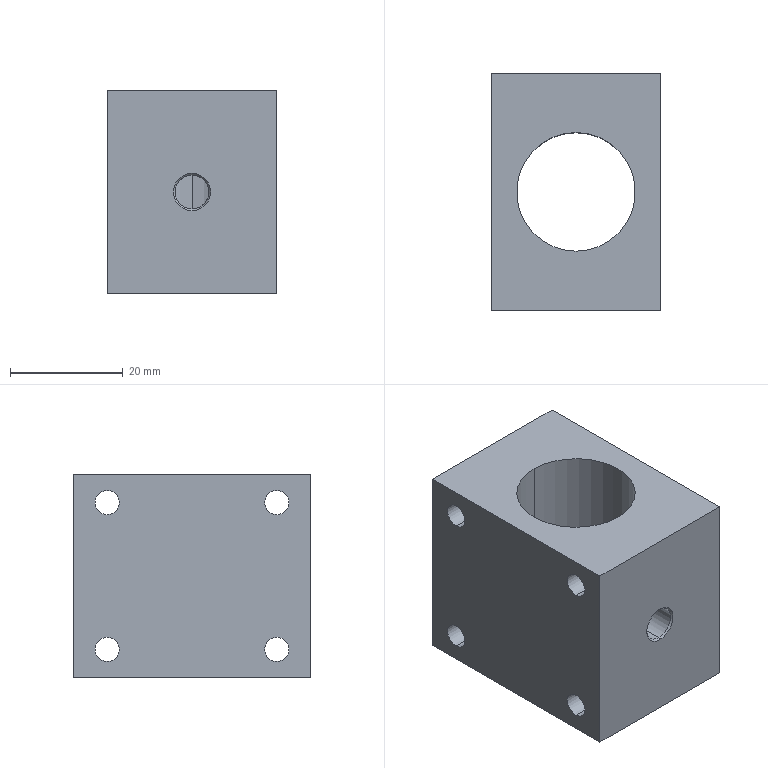Component | SolidWorks | FilmMechanism-3-1_SCLinearBearing-2 | 1 solid | 20 faces | box 30 x 42 x 36 mm | volume 30848 mm3 | cylinder 12 | plane 6 | cone 2 | commonest cylinder face diameters 4.3 x8 6 x2 21 x2
STEP:
#1=COLOUR_RGB('',0.7922,0.8196,0.9333);
#2=FILL_AREA_STYLE_COLOUR('',#1);
#3=FILL_AREA_STYLE('',(#2));
#4=SURFACE_STYLE_FILL_AREA(#3);
#5=SURFACE_SIDE_STYLE('',(#4));
#6=SURFACE_STYLE_USAGE(.BOTH.,#5);
#7=PRESENTATION_STYLE_ASSIGNMENT((#6));
#8=CARTESIAN_POINT('',(-20.718,18.334,-6.681));
#9=VERTEX_POINT('',#8);
#10=CARTESIAN_POINT('',(-20.718,18.334,-6.918));
#11=VERTEX_POINT('',#10);
#12=CARTESIAN_POINT('',(-20.718,18.334,-6.799));
#13=DIRECTION('',(0.,-1.,-0.));
#14=DIRECTION('',(0.,0.,-1.));
#15=AXIS2_PLACEMENT_3D('',#12,#13,#14);
#16=CIRCLE('',#15,0.1181);
#17=EDGE_CURVE('',#9,#11,#16,.T.);
#18=ORIENTED_EDGE('',*,*,#17,.F.);
#19=CARTESIAN_POINT('',(-20.718,18.322,-6.67));
#20=VERTEX_POINT('',#19);
#21=CARTESIAN_POINT('',(-20.718,18.322,-6.67));
#22=DIRECTION('',(0.,-0.7071,0.7071));
#23=VECTOR('',#22,39.37);
#24=LINE('',#21,#23);
#25=EDGE_CURVE('',#9,#20,#24,.T.);
#26=ORIENTED_EDGE('',*,*,#25,.T.);
#27=CARTESIAN_POINT('',(-20.718,18.322,-6.929));
#28=VERTEX_POINT('',#27);
#29=CARTESIAN_POINT('',(-20.718,18.322,-6.799));
#30=DIRECTION('',(0.,-1.,-0.));
#31=DIRECTION('',(0.,0.,-1.));
#32=AXIS2_PLACEMENT_3D('',#29,#30,#31);
#33=CIRCLE('',#32,0.1299);
#34=EDGE_CURVE('',#20,#28,#33,.T.);
#35=ORIENTED_EDGE('',*,*,#34,.T.);
#36=CARTESIAN_POINT('',(-20.718,18.322,-6.929));
#37=DIRECTION('',(0.,-0.7071,-0.7071));
#38=VECTOR('',#37,39.37);
#39=LINE('',#36,#38);
#40=EDGE_CURVE('',#11,#28,#39,.T.);
#41=ORIENTED_EDGE('',*,*,#40,.F.);
#42=EDGE_LOOP('',(#18,#26,#35,#41));
#43=FACE_OUTER_BOUND('',#42,.T.);
#44=CARTESIAN_POINT('',(-20.718,18.322,-6.799));
#45=DIRECTION('',(0.,-1.,-0.));
#46=DIRECTION('',(0.,0.,-1.));
#47=AXIS2_PLACEMENT_3D('',#44,#45,#46);
#48=CONICAL_SURFACE('',#47,0.1299,0.7854);
#49=ADVANCED_FACE('',(#43),#48,.F.);
#50=CARTESIAN_POINT('',(-20.718,18.735,-6.681));
#51=VERTEX_POINT('',#50);
#52=CARTESIAN_POINT('',(-20.718,18.735,-6.918));
#53=VERTEX_POINT('',#52);
#54=CARTESIAN_POINT('',(-20.718,18.735,-6.681));
#55=CARTESIAN_POINT('',(-20.726,18.735,-6.681));
#56=CARTESIAN_POINT('',(-20.734,18.735,-6.682));
#57=CARTESIAN_POINT('',(-20.749,18.736,-6.685));
#58=CARTESIAN_POINT('',(-20.757,18.737,-6.687));
#59=CARTESIAN_POINT('',(-20.771,18.738,-6.693));
#60=CARTESIAN_POINT('',(-20.778,18.739,-6.697));
#61=CARTESIAN_POINT('',(-20.79,18.741,-6.706));
#62=CARTESIAN_POINT('',(-20.796,18.743,-6.71));
#63=CARTESIAN_POINT('',(-20.807,18.745,-6.721));
#64=CARTESIAN_POINT('',(-20.812,18.746,-6.727));
#65=CARTESIAN_POINT('',(-20.821,18.748,-6.74));
#66=CARTESIAN_POINT('',(-20.824,18.749,-6.747));
#67=CARTESIAN_POINT('',(-20.83,18.751,-6.761));
#68=CARTESIAN_POINT('',(-20.833,18.751,-6.769));
#69=CARTESIAN_POINT('',(-20.836,18.752,-6.784));
#70=CARTESIAN_POINT('',(-20.836,18.752,-6.792));
#71=CARTESIAN_POINT('',(-20.836,18.752,-6.807));
#72=CARTESIAN_POINT('',(-20.836,18.752,-6.815));
#73=CARTESIAN_POINT('',(-20.833,18.751,-6.83));
#74=CARTESIAN_POINT('',(-20.83,18.751,-6.838));
#75=CARTESIAN_POINT('',(-20.822,18.748,-6.859));
#76=CARTESIAN_POINT('',(-20.813,18.746,-6.872));
#77=CARTESIAN_POINT('',(-20.797,18.743,-6.888));
#78=CARTESIAN_POINT('',(-20.79,18.741,-6.893));
#79=CARTESIAN_POINT('',(-20.778,18.739,-6.902));
#80=CARTESIAN_POINT('',(-20.771,18.738,-6.906));
#81=CARTESIAN_POINT('',(-20.757,18.737,-6.911));
#82=CARTESIAN_POINT('',(-20.749,18.736,-6.914));
#83=CARTESIAN_POINT('',(-20.734,18.735,-6.917));
#84=CARTESIAN_POINT('',(-20.726,18.735,-6.918));
#85=CARTESIAN_POINT('',(-20.718,18.735,-6.918));
#86=B_SPLINE_CURVE_WITH_KNOTS('',3,(#54,#55,#56,#57,#58,#59,#60,#61,#62,#63,#64,#65,#66,#67,#68,#69,#70,#71,#72,#73,#74,#75,#76,#77,#78,#79,#80,#81,#82,#83,#84,#85),.UNSPECIFIED.,.F.,.F.,(4,2,2,2,2,2,2,2,2,2,2,2,2,2,2,4),(0.009429,0.01002,0.01061,0.0112,0.01179,0.01237,0.01296,0.01355,0.01414,0.01473,0.01532,0.0165,0.01709,0.01768,0.01827,0.01885),.UNSPECIFIED.);
#87=EDGE_CURVE('',#51,#53,#86,.T.);
#88=ORIENTED_EDGE('',*,*,#87,.F.);
#89=CARTESIAN_POINT('',(-20.718,18.322,-6.681));
#90=DIRECTION('',(0.,-1.,-0.));
#91=VECTOR('',#90,39.37);
#92=LINE('',#89,#91);
#93=EDGE_CURVE('',#51,#9,#92,.T.);
#94=ORIENTED_EDGE('',*,*,#93,.T.);
#95=ORIENTED_EDGE('',*,*,#17,.T.);
#96=CARTESIAN_POINT('',(-20.718,18.322,-6.918));
#97=DIRECTION('',(0.,-1.,-0.));
#98=VECTOR('',#97,39.37);
#99=LINE('',#96,#98);
#100=EDGE_CURVE('',#53,#11,#99,.T.);
#101=ORIENTED_EDGE('',*,*,#100,.F.);
#102=EDGE_LOOP('',(#88,#94,#95,#101));
#103=FACE_OUTER_BOUND('',#102,.T.);
#104=CARTESIAN_POINT('',(-20.718,18.322,-6.799));
#105=DIRECTION('',(0.,-1.,-0.));
#106=DIRECTION('',(0.,0.,-1.));
#107=AXIS2_PLACEMENT_3D('',#104,#105,#106);
#108=CYLINDRICAL_SURFACE('',#107,0.1181);
#109=ADVANCED_FACE('',(#103),#108,.F.);
#110=CARTESIAN_POINT('',(-20.718,19.562,-7.508));
#111=VERTEX_POINT('',#110);
#112=CARTESIAN_POINT('',(-20.718,18.735,-7.508));
#113=VERTEX_POINT('',#112);
#114=CARTESIAN_POINT('',(-20.718,19.149,-7.508));
#115=DIRECTION('',(-0.,-0.,1.));
#116=DIRECTION('',(0.,-1.,-0.));
#117=AXIS2_PLACEMENT_3D('',#114,#115,#116);
#118=CIRCLE('',#117,0.4134);
#119=EDGE_CURVE('',#111,#113,#118,.T.);
#120=ORIENTED_EDGE('',*,*,#119,.F.);
#121=CARTESIAN_POINT('',(-20.718,19.562,-6.091));
#122=VERTEX_POINT('',#121);
#123=CARTESIAN_POINT('',(-20.718,19.562,-6.091));
#124=DIRECTION('',(-0.,-0.,1.));
#125=VECTOR('',#124,39.37);
#126=LINE('',#123,#125);
#127=EDGE_CURVE('',#111,#122,#126,.T.);
#128=ORIENTED_EDGE('',*,*,#127,.T.);
#129=CARTESIAN_POINT('',(-20.718,18.735,-6.091));
#130=VERTEX_POINT('',#129);
#131=CARTESIAN_POINT('',(-20.718,19.149,-6.091));
#132=DIRECTION('',(-0.,-0.,1.));
#133=DIRECTION('',(0.,-1.,-0.));
#134=AXIS2_PLACEMENT_3D('',#131,#132,#133);
#135=CIRCLE('',#134,0.4134);
#136=EDGE_CURVE('',#122,#130,#135,.T.);
#137=ORIENTED_EDGE('',*,*,#136,.T.);
#138=CARTESIAN_POINT('',(-20.718,18.735,-6.091));
#139=DIRECTION('',(-0.,-0.,1.));
#140=VECTOR('',#139,39.37);
#141=LINE('',#138,#140);
#142=EDGE_CURVE('',#51,#130,#141,.T.);
#143=ORIENTED_EDGE('',*,*,#142,.F.);
#144=ORIENTED_EDGE('',*,*,#87,.T.);
#145=CARTESIAN_POINT('',(-20.718,18.735,-6.091));
#146=DIRECTION('',(-0.,-0.,1.));
#147=VECTOR('',#146,39.37);
#148=LINE('',#145,#147);
#149=EDGE_CURVE('',#113,#53,#148,.T.);
#150=ORIENTED_EDGE('',*,*,#149,.F.);
#151=EDGE_LOOP('',(#120,#128,#137,#143,#144,#150));
#152=FACE_OUTER_BOUND('',#151,.T.);
#153=CARTESIAN_POINT('',(-20.718,19.149,-6.091));
#154=DIRECTION('',(-0.,-0.,1.));
#155=DIRECTION('',(0.,-1.,-0.));
#156=AXIS2_PLACEMENT_3D('',#153,#154,#155);
#157=CYLINDRICAL_SURFACE('',#156,0.4134);
#158=ADVANCED_FACE('',(#152),#157,.F.);
#159=CARTESIAN_POINT('',(-20.128,19.739,-7.227));
#160=VERTEX_POINT('',#159);
#161=CARTESIAN_POINT('',(-20.128,19.739,-7.396));
#162=VERTEX_POINT('',#161);
#163=CARTESIAN_POINT('',(-20.128,19.739,-7.311));
#164=DIRECTION('',(-1.,-0.,-0.));
#165=DIRECTION('',(0.,0.,-1.));
#166=AXIS2_PLACEMENT_3D('',#163,#164,#165);
#167=CIRCLE('',#166,0.08465);
#168=EDGE_CURVE('',#160,#162,#167,.T.);
#169=ORIENTED_EDGE('',*,*,#168,.F.);
#170=CARTESIAN_POINT('',(-21.309,19.739,-7.227));
#171=VERTEX_POINT('',#170);
#172=CARTESIAN_POINT('',(-21.309,19.739,-7.227));
#173=DIRECTION('',(-1.,-0.,-0.));
#174=VECTOR('',#173,39.37);
#175=LINE('',#172,#174);
#176=EDGE_CURVE('',#160,#171,#175,.T.);
#177=ORIENTED_EDGE('',*,*,#176,.T.);
#178=CARTESIAN_POINT('',(-21.309,19.739,-7.396));
#179=VERTEX_POINT('',#178);
#180=CARTESIAN_POINT('',(-21.309,19.739,-7.311));
#181=DIRECTION('',(-1.,-0.,-0.));
#182=DIRECTION('',(0.,0.,-1.));
#183=AXIS2_PLACEMENT_3D('',#180,#181,#182);
#184=CIRCLE('',#183,0.08465);
#185=EDGE_CURVE('',#171,#179,#184,.T.);
#186=ORIENTED_EDGE('',*,*,#185,.T.);
#187=CARTESIAN_POINT('',(-21.309,19.739,-7.396));
#188=DIRECTION('',(-1.,-0.,-0.));
#189=VECTOR('',#188,39.37);
#190=LINE('',#187,#189);
#191=EDGE_CURVE('',#162,#179,#190,.T.);
#192=ORIENTED_EDGE('',*,*,#191,.F.);
#193=EDGE_LOOP('',(#169,#177,#186,#192));
#194=FACE_OUTER_BOUND('',#193,.T.);
#195=CARTESIAN_POINT('',(-21.309,19.739,-7.311));
#196=DIRECTION('',(-1.,-0.,-0.));
#197=DIRECTION('',(0.,0.,-1.));
#198=AXIS2_PLACEMENT_3D('',#195,#196,#197);
#199=CYLINDRICAL_SURFACE('',#198,0.08465);
#200=ADVANCED_FACE('',(#194),#199,.F.);
#201=CARTESIAN_POINT('',(-20.128,19.739,-6.203));
#202=VERTEX_POINT('',#201);
#203=CARTESIAN_POINT('',(-20.128,19.739,-6.372));
#204=VERTEX_POINT('',#203);
#205=CARTESIAN_POINT('',(-20.128,19.739,-6.288));
#206=DIRECTION('',(-1.,-0.,-0.));
#207=DIRECTION('',(0.,0.,-1.));
#208=AXIS2_PLACEMENT_3D('',#205,#206,#207);
#209=CIRCLE('',#208,0.08465);
#210=EDGE_CURVE('',#202,#204,#209,.T.);
#211=ORIENTED_EDGE('',*,*,#210,.F.);
#212=CARTESIAN_POINT('',(-21.309,19.739,-6.203));
#213=VERTEX_POINT('',#212);
#214=CARTESIAN_POINT('',(-21.309,19.739,-6.203));
#215=DIRECTION('',(-1.,-0.,-0.));
#216=VECTOR('',#215,39.37);
#217=LINE('',#214,#216);
#218=EDGE_CURVE('',#202,#213,#217,.T.);
#219=ORIENTED_EDGE('',*,*,#218,.T.);
#220=CARTESIAN_POINT('',(-21.309,19.739,-6.372));
#221=VERTEX_POINT('',#220);
#222=CARTESIAN_POINT('',(-21.309,19.739,-6.288));
#223=DIRECTION('',(-1.,-0.,-0.));
#224=DIRECTION('',(0.,0.,-1.));
#225=AXIS2_PLACEMENT_3D('',#222,#223,#224);
#226=CIRCLE('',#225,0.08465);
#227=EDGE_CURVE('',#213,#221,#226,.T.);
#228=ORIENTED_EDGE('',*,*,#227,.T.);
#229=CARTESIAN_POINT('',(-21.309,19.739,-6.372));
#230=DIRECTION('',(-1.,-0.,-0.));
#231=VECTOR('',#230,39.37);
#232=LINE('',#229,#231);
#233=EDGE_CURVE('',#204,#221,#232,.T.);
#234=ORIENTED_EDGE('',*,*,#233,.F.);
#235=EDGE_LOOP('',(#211,#219,#228,#234));
#236=FACE_OUTER_BOUND('',#235,.T.);
#237=CARTESIAN_POINT('',(-21.309,19.739,-6.288));
#238=DIRECTION('',(-1.,-0.,-0.));
#239=DIRECTION('',(0.,0.,-1.));
#240=AXIS2_PLACEMENT_3D('',#237,#238,#239);
#241=CYLINDRICAL_SURFACE('',#240,0.08465);
#242=ADVANCED_FACE('',(#236),#241,.F.);
#243=CARTESIAN_POINT('',(-20.128,18.558,-7.227));
#244=VERTEX_POINT('',#243);
#245=CARTESIAN_POINT('',(-20.128,18.558,-7.396));
#246=VERTEX_POINT('',#245);
#247=CARTESIAN_POINT('',(-20.128,18.558,-7.311));
#248=DIRECTION('',(-1.,-0.,-0.));
#249=DIRECTION('',(0.,0.,-1.));
#250=AXIS2_PLACEMENT_3D('',#247,#248,#249);
#251=CIRCLE('',#250,0.08465);
#252=EDGE_CURVE('',#244,#246,#251,.T.);
#253=ORIENTED_EDGE('',*,*,#252,.F.);
#254=CARTESIAN_POINT('',(-21.309,18.558,-7.227));
#255=VERTEX_POINT('',#254);
#256=CARTESIAN_POINT('',(-21.309,18.558,-7.227));
#257=DIRECTION('',(-1.,-0.,-0.));
#258=VECTOR('',#257,39.37);
#259=LINE('',#256,#258);
#260=EDGE_CURVE('',#244,#255,#259,.T.);
#261=ORIENTED_EDGE('',*,*,#260,.T.);
#262=CARTESIAN_POINT('',(-21.309,18.558,-7.396));
#263=VERTEX_POINT('',#262);
#264=CARTESIAN_POINT('',(-21.309,18.558,-7.311));
#265=DIRECTION('',(-1.,-0.,-0.));
#266=DIRECTION('',(0.,0.,-1.));
#267=AXIS2_PLACEMENT_3D('',#264,#265,#266);
#268=CIRCLE('',#267,0.08465);
#269=EDGE_CURVE('',#255,#263,#268,.T.);
#270=ORIENTED_EDGE('',*,*,#269,.T.);
#271=CARTESIAN_POINT('',(-21.309,18.558,-7.396));
#272=DIRECTION('',(-1.,-0.,-0.));
#273=VECTOR('',#272,39.37);
#274=LINE('',#271,#273);
#275=EDGE_CURVE('',#246,#263,#274,.T.);
#276=ORIENTED_EDGE('',*,*,#275,.F.);
#277=EDGE_LOOP('',(#253,#261,#270,#276));
#278=FACE_OUTER_BOUND('',#277,.T.);
#279=CARTESIAN_POINT('',(-21.309,18.558,-7.311));
#280=DIRECTION('',(-1.,-0.,-0.));
#281=DIRECTION('',(0.,0.,-1.));
#282=AXIS2_PLACEMENT_3D('',#279,#280,#281);
#283=CYLINDRICAL_SURFACE('',#282,0.08465);
#284=ADVANCED_FACE('',(#278),#283,.F.);
#285=CARTESIAN_POINT('',(-20.128,18.558,-6.203));
#286=VERTEX_POINT('',#285);
#287=CARTESIAN_POINT('',(-20.128,18.558,-6.372));
#288=VERTEX_POINT('',#287);
#289=CARTESIAN_POINT('',(-20.128,18.558,-6.288));
#290=DIRECTION('',(-1.,-0.,-0.));
#291=DIRECTION('',(0.,0.,-1.));
#292=AXIS2_PLACEMENT_3D('',#289,#290,#291);
#293=CIRCLE('',#292,0.08465);
#294=EDGE_CURVE('',#286,#288,#293,.T.);
#295=ORIENTED_EDGE('',*,*,#294,.F.);
#296=CARTESIAN_POINT('',(-21.309,18.558,-6.203));
#297=VERTEX_POINT('',#296);
#298=CARTESIAN_POINT('',(-21.309,18.558,-6.203));
#299=DIRECTION('',(-1.,-0.,-0.));
#300=VECTOR('',#299,39.37);
#301=LINE('',#298,#300);
#302=EDGE_CURVE('',#286,#297,#301,.T.);
#303=ORIENTED_EDGE('',*,*,#302,.T.);
#304=CARTESIAN_POINT('',(-21.309,18.558,-6.372));
#305=VERTEX_POINT('',#304);
#306=CARTESIAN_POINT('',(-21.309,18.558,-6.288));
#307=DIRECTION('',(-1.,-0.,-0.));
#308=DIRECTION('',(0.,0.,-1.));
#309=AXIS2_PLACEMENT_3D('',#306,#307,#308);
#310=CIRCLE('',#309,0.08465);
#311=EDGE_CURVE('',#297,#305,#310,.T.);
#312=ORIENTED_EDGE('',*,*,#311,.T.);
#313=CARTESIAN_POINT('',(-21.309,18.558,-6.372));
#314=DIRECTION('',(-1.,-0.,-0.));
#315=VECTOR('',#314,39.37);
#316=LINE('',#313,#315);
#317=EDGE_CURVE('',#288,#305,#316,.T.);
#318=ORIENTED_EDGE('',*,*,#317,.F.);
#319=EDGE_LOOP('',(#295,#303,#312,#318));
#320=FACE_OUTER_BOUND('',#319,.T.);
#321=CARTESIAN_POINT('',(-21.309,18.558,-6.288));
#322=DIRECTION('',(-1.,-0.,-0.));
#323=DIRECTION('',(0.,0.,-1.));
#324=AXIS2_PLACEMENT_3D('',#321,#322,#323);
#325=CYLINDRICAL_SURFACE('',#324,0.08465);
#326=ADVANCED_FACE('',(#320),#325,.F.);
#327=CARTESIAN_POINT('',(-20.718,18.322,-6.799));
#328=DIRECTION('',(0.,-1.,-0.));
#329=DIRECTION('',(0.,0.,-1.));
#330=AXIS2_PLACEMENT_3D('',#327,#328,#329);
#331=CIRCLE('',#330,0.1299);
#332=EDGE_CURVE('',#28,#20,#331,.T.);
#333=ORIENTED_EDGE('',*,*,#332,.F.);
#334=ORIENTED_EDGE('',*,*,#34,.F.);
#335=EDGE_LOOP('',(#333,#334));
#336=FACE_BOUND('',#335,.T.);
#337=CARTESIAN_POINT('',(-21.309,18.322,-7.508));
#338=VERTEX_POINT('',#337);
#339=CARTESIAN_POINT('',(-21.309,18.322,-6.091));
#340=VERTEX_POINT('',#339);
#341=CARTESIAN_POINT('',(-21.309,18.322,-7.508));
#342=DIRECTION('',(-0.,-0.,1.));
#343=VECTOR('',#342,39.37);
#344=LINE('',#341,#343);
#345=EDGE_CURVE('',#338,#340,#344,.T.);
#346=ORIENTED_EDGE('',*,*,#345,.F.);
#347=CARTESIAN_POINT('',(-20.128,18.322,-7.508));
#348=VERTEX_POINT('',#347);
#349=CARTESIAN_POINT('',(-20.128,18.322,-7.508));
#350=DIRECTION('',(-1.,-0.,-0.));
#351=VECTOR('',#350,39.37);
#352=LINE('',#349,#351);
#353=EDGE_CURVE('',#348,#338,#352,.T.);
#354=ORIENTED_EDGE('',*,*,#353,.F.);
#355=CARTESIAN_POINT('',(-20.128,18.322,-6.091));
#356=VERTEX_POINT('',#355);
#357=CARTESIAN_POINT('',(-20.128,18.322,-7.508));
#358=DIRECTION('',(-0.,-0.,1.));
#359=VECTOR('',#358,39.37);
#360=LINE('',#357,#359);
#361=EDGE_CURVE('',#348,#356,#360,.T.);
#362=ORIENTED_EDGE('',*,*,#361,.T.);
#363=CARTESIAN_POINT('',(-20.128,18.322,-6.091));
#364=DIRECTION('',(-1.,-0.,-0.));
#365=VECTOR('',#364,39.37);
#366=LINE('',#363,#365);
#367=EDGE_CURVE('',#356,#340,#366,.T.);
#368=ORIENTED_EDGE('',*,*,#367,.T.);
#369=EDGE_LOOP('',(#346,#354,#362,#368));
#370=FACE_OUTER_BOUND('',#369,.T.);
#371=CARTESIAN_POINT('',(-20.128,18.322,-7.508));
#372=DIRECTION('',(0.,-1.,-0.));
#373=DIRECTION('',(0.,0.,-1.));
#374=AXIS2_PLACEMENT_3D('',#371,#372,#373);
#375=PLANE('',#374);
#376=ADVANCED_FACE('',(#336,#370),#375,.T.);
#377=CARTESIAN_POINT('',(-20.718,19.149,-7.508));
#378=DIRECTION('',(-0.,-0.,1.));
#379=DIRECTION('',(0.,-1.,-0.));
#380=AXIS2_PLACEMENT_3D('',#377,#378,#379);
#381=CIRCLE('',#380,0.4134);
#382=EDGE_CURVE('',#113,#111,#381,.T.);
#383=ORIENTED_EDGE('',*,*,#382,.T.);
#384=ORIENTED_EDGE('',*,*,#119,.T.);
#385=EDGE_LOOP('',(#383,#384));
#386=FACE_BOUND('',#385,.T.);
#387=CARTESIAN_POINT('',(-21.309,19.975,-7.508));
#388=VERTEX_POINT('',#387);
#389=CARTESIAN_POINT('',(-21.309,19.975,-7.508));
#390=DIRECTION('',(0.,-1.,-0.));
#391=VECTOR('',#390,39.37);
#392=LINE('',#389,#391);
#393=EDGE_CURVE('',#388,#338,#392,.T.);
#394=ORIENTED_EDGE('',*,*,#393,.F.);
#395=CARTESIAN_POINT('',(-20.128,19.975,-7.508));
#396=VERTEX_POINT('',#395);
#397=CARTESIAN_POINT('',(-20.128,19.975,-7.508));
#398=DIRECTION('',(-1.,-0.,-0.));
#399=VECTOR('',#398,39.37);
#400=LINE('',#397,#399);
#401=EDGE_CURVE('',#396,#388,#400,.T.);
#402=ORIENTED_EDGE('',*,*,#401,.F.);
#403=CARTESIAN_POINT('',(-20.128,19.975,-7.508));
#404=DIRECTION('',(0.,-1.,-0.));
#405=VECTOR('',#404,39.37);
#406=LINE('',#403,#405);
#407=EDGE_CURVE('',#396,#348,#406,.T.);
#408=ORIENTED_EDGE('',*,*,#407,.T.);
#409=ORIENTED_EDGE('',*,*,#353,.T.);
#410=EDGE_LOOP('',(#394,#402,#408,#409));
#411=FACE_OUTER_BOUND('',#410,.T.);
#412=CARTESIAN_POINT('',(-20.128,19.975,-7.508));
#413=DIRECTION('',(0.,0.,-1.));
#414=DIRECTION('',(-0.,1.,0.));
#415=AXIS2_PLACEMENT_3D('',#412,#413,#414);
#416=PLANE('',#415);
#417=ADVANCED_FACE('',(#386,#411),#416,.T.);
#418=CARTESIAN_POINT('',(-21.309,19.975,-6.091));
#419=VERTEX_POINT('',#418);
#420=CARTESIAN_POINT('',(-21.309,19.975,-6.091));
#421=DIRECTION('',(0.,0.,-1.));
#422=VECTOR('',#421,39.37);
#423=LINE('',#420,#422);
#424=EDGE_CURVE('',#419,#388,#423,.T.);
#425=ORIENTED_EDGE('',*,*,#424,.F.);
#426=CARTESIAN_POINT('',(-20.128,19.975,-6.091));
#427=VERTEX_POINT('',#426);
#428=CARTESIAN_POINT('',(-20.128,19.975,-6.091));
#429=DIRECTION('',(-1.,-0.,-0.));
#430=VECTOR('',#429,39.37);
#431=LINE('',#428,#430);
#432=EDGE_CURVE('',#427,#419,#431,.T.);
#433=ORIENTED_EDGE('',*,*,#432,.F.);
#434=CARTESIAN_POINT('',(-20.128,19.975,-6.091));
#435=DIRECTION('',(0.,0.,-1.));
#436=VECTOR('',#435,39.37);
#437=LINE('',#434,#436);
#438=EDGE_CURVE('',#427,#396,#437,.T.);
#439=ORIENTED_EDGE('',*,*,#438,.T.);
#440=ORIENTED_EDGE('',*,*,#401,.T.);
#441=EDGE_LOOP('',(#425,#433,#439,#440));
#442=FACE_OUTER_BOUND('',#441,.T.);
#443=CARTESIAN_POINT('',(-20.128,19.975,-6.091));
#444=DIRECTION('',(-0.,1.,0.));
#445=DIRECTION('',(-0.,-0.,1.));
#446=AXIS2_PLACEMENT_3D('',#443,#444,#445);
#447=PLANE('',#446);
#448=ADVANCED_FACE('',(#442),#447,.T.);
#449=CARTESIAN_POINT('',(-20.718,19.149,-6.091));
#450=DIRECTION('',(-0.,-0.,1.));
#451=DIRECTION('',(0.,-1.,-0.));
#452=AXIS2_PLACEMENT_3D('',#449,#450,#451);
#453=CIRCLE('',#452,0.4134);
#454=EDGE_CURVE('',#130,#122,#453,.T.);
#455=ORIENTED_EDGE('',*,*,#454,.F.);
#456=ORIENTED_EDGE('',*,*,#136,.F.);
#457=EDGE_LOOP('',(#455,#456));
#458=FACE_BOUND('',#457,.T.);
#459=CARTESIAN_POINT('',(-21.309,18.322,-6.091));
#460=DIRECTION('',(-0.,1.,0.));
#461=VECTOR('',#460,39.37);
#462=LINE('',#459,#461);
#463=EDGE_CURVE('',#340,#419,#462,.T.);
#464=ORIENTED_EDGE('',*,*,#463,.F.);
#465=ORIENTED_EDGE('',*,*,#367,.F.);
#466=CARTESIAN_POINT('',(-20.128,18.322,-6.091));
#467=DIRECTION('',(-0.,1.,0.));
#468=VECTOR('',#467,39.37);
#469=LINE('',#466,#468);
#470=EDGE_CURVE('',#356,#427,#469,.T.);
#471=ORIENTED_EDGE('',*,*,#470,.T.);
#472=ORIENTED_EDGE('',*,*,#432,.T.);
#473=EDGE_LOOP('',(#464,#465,#471,#472));
#474=FACE_OUTER_BOUND('',#473,.T.);
#475=CARTESIAN_POINT('',(-20.128,18.322,-6.091));
#476=DIRECTION('',(-0.,-0.,1.));
#477=DIRECTION('',(0.,-1.,-0.));
#478=AXIS2_PLACEMENT_3D('',#475,#476,#477);
#479=PLANE('',#478);
#480=ADVANCED_FACE('',(#458,#474),#479,.T.);
#481=CARTESIAN_POINT('',(-20.128,19.739,-7.311));
#482=DIRECTION('',(-1.,-0.,-0.));
#483=DIRECTION('',(0.,0.,-1.));
#484=AXIS2_PLACEMENT_3D('',#481,#482,#483);
#485=CIRCLE('',#484,0.08465);
#486=EDGE_CURVE('',#162,#160,#485,.T.);
#487=ORIENTED_EDGE('',*,*,#486,.T.);
#488=ORIENTED_EDGE('',*,*,#168,.T.);
#489=EDGE_LOOP('',(#487,#488));
#490=FACE_BOUND('',#489,.T.);
#491=CARTESIAN_POINT('',(-20.128,19.739,-6.288));
#492=DIRECTION('',(-1.,-0.,-0.));
#493=DIRECTION('',(0.,0.,-1.));
#494=AXIS2_PLACEMENT_3D('',#491,#492,#493);
#495=CIRCLE('',#494,0.08465);
#496=EDGE_CURVE('',#204,#202,#495,.T.);
#497=ORIENTED_EDGE('',*,*,#496,.T.);
#498=ORIENTED_EDGE('',*,*,#210,.T.);
#499=EDGE_LOOP('',(#497,#498));
#500=FACE_BOUND('',#499,.T.);
#501=CARTESIAN_POINT('',(-20.128,18.558,-7.311));
#502=DIRECTION('',(-1.,-0.,-0.));
#503=DIRECTION('',(0.,0.,-1.));
#504=AXIS2_PLACEMENT_3D('',#501,#502,#503);
#505=CIRCLE('',#504,0.08465);
#506=EDGE_CURVE('',#246,#244,#505,.T.);
#507=ORIENTED_EDGE('',*,*,#506,.T.);
#508=ORIENTED_EDGE('',*,*,#252,.T.);
#509=EDGE_LOOP('',(#507,#508));
#510=FACE_BOUND('',#509,.T.);
#511=CARTESIAN_POINT('',(-20.128,18.558,-6.288));
#512=DIRECTION('',(-1.,-0.,-0.));
#513=DIRECTION('',(0.,0.,-1.));
#514=AXIS2_PLACEMENT_3D('',#511,#512,#513);
#515=CIRCLE('',#514,0.08465);
#516=EDGE_CURVE('',#288,#286,#515,.T.);
#517=ORIENTED_EDGE('',*,*,#516,.T.);
#518=ORIENTED_EDGE('',*,*,#294,.T.);
#519=EDGE_LOOP('',(#517,#518));
#520=FACE_BOUND('',#519,.T.);
#521=ORIENTED_EDGE('',*,*,#361,.F.);
#522=ORIENTED_EDGE('',*,*,#407,.F.);
#523=ORIENTED_EDGE('',*,*,#438,.F.);
#524=ORIENTED_EDGE('',*,*,#470,.F.);
#525=EDGE_LOOP('',(#521,#522,#523,#524));
#526=FACE_OUTER_BOUND('',#525,.T.);
#527=CARTESIAN_POINT('',(-20.128,19.149,-6.799));
#528=DIRECTION('',(-1.,-0.,-0.));
#529=DIRECTION('',(0.,0.,-1.));
#530=AXIS2_PLACEMENT_3D('',#527,#528,#529);
#531=PLANE('',#530);
#532=ADVANCED_FACE('',(#490,#500,#510,#520,#526),#531,.F.);
#533=CARTESIAN_POINT('',(-21.309,19.739,-7.311));
#534=DIRECTION('',(-1.,-0.,-0.));
#535=DIRECTION('',(0.,0.,-1.));
#536=AXIS2_PLACEMENT_3D('',#533,#534,#535);
#537=CIRCLE('',#536,0.08465);
#538=EDGE_CURVE('',#179,#171,#537,.T.);
#539=ORIENTED_EDGE('',*,*,#538,.F.);
#540=ORIENTED_EDGE('',*,*,#185,.F.);
#541=EDGE_LOOP('',(#539,#540));
#542=FACE_BOUND('',#541,.T.);
#543=CARTESIAN_POINT('',(-21.309,19.739,-6.288));
#544=DIRECTION('',(-1.,-0.,-0.));
#545=DIRECTION('',(0.,0.,-1.));
#546=AXIS2_PLACEMENT_3D('',#543,#544,#545);
#547=CIRCLE('',#546,0.08465);
#548=EDGE_CURVE('',#221,#213,#547,.T.);
#549=ORIENTED_EDGE('',*,*,#548,.F.);
#550=ORIENTED_EDGE('',*,*,#227,.F.);
#551=EDGE_LOOP('',(#549,#550));
#552=FACE_BOUND('',#551,.T.);
#553=CARTESIAN_POINT('',(-21.309,18.558,-7.311));
#554=DIRECTION('',(-1.,-0.,-0.));
#555=DIRECTION('',(0.,0.,-1.));
#556=AXIS2_PLACEMENT_3D('',#553,#554,#555);
#557=CIRCLE('',#556,0.08465);
#558=EDGE_CURVE('',#263,#255,#557,.T.);
#559=ORIENTED_EDGE('',*,*,#558,.F.);
#560=ORIENTED_EDGE('',*,*,#269,.F.);
#561=EDGE_LOOP('',(#559,#560));
#562=FACE_BOUND('',#561,.T.);
#563=CARTESIAN_POINT('',(-21.309,18.558,-6.288));
#564=DIRECTION('',(-1.,-0.,-0.));
#565=DIRECTION('',(0.,0.,-1.));
#566=AXIS2_PLACEMENT_3D('',#563,#564,#565);
#567=CIRCLE('',#566,0.08465);
#568=EDGE_CURVE('',#305,#297,#567,.T.);
#569=ORIENTED_EDGE('',*,*,#568,.F.);
#570=ORIENTED_EDGE('',*,*,#311,.F.);
#571=EDGE_LOOP('',(#569,#570));
#572=FACE_BOUND('',#571,.T.);
#573=ORIENTED_EDGE('',*,*,#345,.T.);
#574=ORIENTED_EDGE('',*,*,#463,.T.);
#575=ORIENTED_EDGE('',*,*,#424,.T.);
#576=ORIENTED_EDGE('',*,*,#393,.T.);
#577=EDGE_LOOP('',(#573,#574,#575,#576));
#578=FACE_OUTER_BOUND('',#577,.T.);
#579=CARTESIAN_POINT('',(-21.309,19.149,-6.799));
#580=DIRECTION('',(-1.,-0.,-0.));
#581=DIRECTION('',(0.,0.,-1.));
#582=AXIS2_PLACEMENT_3D('',#579,#580,#581);
#583=PLANE('',#582);
#584=ADVANCED_FACE('',(#542,#552,#562,#572,#578),#583,.T.);
#585=ORIENTED_EDGE('',*,*,#302,.F.);
#586=ORIENTED_EDGE('',*,*,#516,.F.);
#587=ORIENTED_EDGE('',*,*,#317,.T.);
#588=ORIENTED_EDGE('',*,*,#568,.T.);
#589=EDGE_LOOP('',(#585,#586,#587,#588));
#590=FACE_OUTER_BOUND('',#589,.T.);
#591=CARTESIAN_POINT('',(-21.309,18.558,-6.288));
#592=DIRECTION('',(-1.,-0.,-0.));
#593=DIRECTION('',(0.,0.,-1.));
#594=AXIS2_PLACEMENT_3D('',#591,#592,#593);
#595=CYLINDRICAL_SURFACE('',#594,0.08465);
#596=ADVANCED_FACE('',(#590),#595,.F.);
#597=ORIENTED_EDGE('',*,*,#260,.F.);
#598=ORIENTED_EDGE('',*,*,#506,.F.);
#599=ORIENTED_EDGE('',*,*,#275,.T.);
#600=ORIENTED_EDGE('',*,*,#558,.T.);
#601=EDGE_LOOP('',(#597,#598,#599,#600));
#602=FACE_OUTER_BOUND('',#601,.T.);
#603=CARTESIAN_POINT('',(-21.309,18.558,-7.311));
#604=DIRECTION('',(-1.,-0.,-0.));
#605=DIRECTION('',(0.,0.,-1.));
#606=AXIS2_PLACEMENT_3D('',#603,#604,#605);
#607=CYLINDRICAL_SURFACE('',#606,0.08465);
#608=ADVANCED_FACE('',(#602),#607,.F.);
#609=ORIENTED_EDGE('',*,*,#218,.F.);
#610=ORIENTED_EDGE('',*,*,#496,.F.);
#611=ORIENTED_EDGE('',*,*,#233,.T.);
#612=ORIENTED_EDGE('',*,*,#548,.T.);
#613=EDGE_LOOP('',(#609,#610,#611,#612));
#614=FACE_OUTER_BOUND('',#613,.T.);
#615=CARTESIAN_POINT('',(-21.309,19.739,-6.288));
#616=DIRECTION('',(-1.,-0.,-0.));
#617=DIRECTION('',(0.,0.,-1.));
#618=AXIS2_PLACEMENT_3D('',#615,#616,#617);
#619=CYLINDRICAL_SURFACE('',#618,0.08465);
#620=ADVANCED_FACE('',(#614),#619,.F.);
#621=ORIENTED_EDGE('',*,*,#176,.F.);
#622=ORIENTED_EDGE('',*,*,#486,.F.);
#623=ORIENTED_EDGE('',*,*,#191,.T.);
#624=ORIENTED_EDGE('',*,*,#538,.T.);
#625=EDGE_LOOP('',(#621,#622,#623,#624));
#626=FACE_OUTER_BOUND('',#625,.T.);
#627=CARTESIAN_POINT('',(-21.309,19.739,-7.311));
#628=DIRECTION('',(-1.,-0.,-0.));
#629=DIRECTION('',(0.,0.,-1.));
#630=AXIS2_PLACEMENT_3D('',#627,#628,#629);
#631=CYLINDRICAL_SURFACE('',#630,0.08465);
#632=ADVANCED_FACE('',(#626),#631,.F.);
#633=ORIENTED_EDGE('',*,*,#127,.F.);
#634=ORIENTED_EDGE('',*,*,#382,.F.);
#635=ORIENTED_EDGE('',*,*,#149,.T.);
#636=CARTESIAN_POINT('',(-20.718,18.735,-6.918));
#637=CARTESIAN_POINT('',(-20.711,18.735,-6.918));
#638=CARTESIAN_POINT('',(-20.703,18.735,-6.917));
#639=CARTESIAN_POINT('',(-20.688,18.736,-6.914));
#640=CARTESIAN_POINT('',(-20.68,18.737,-6.911));
#641=CARTESIAN_POINT('',(-20.666,18.738,-6.906));
#642=CARTESIAN_POINT('',(-20.659,18.739,-6.902));
#643=CARTESIAN_POINT('',(-20.646,18.741,-6.893));
#644=CARTESIAN_POINT('',(-20.64,18.743,-6.888));
#645=CARTESIAN_POINT('',(-20.624,18.746,-6.872));
#646=CARTESIAN_POINT('',(-20.615,18.748,-6.859));
#647=CARTESIAN_POINT('',(-20.606,18.751,-6.838));
#648=CARTESIAN_POINT('',(-20.604,18.751,-6.83));
#649=CARTESIAN_POINT('',(-20.601,18.752,-6.815));
#650=CARTESIAN_POINT('',(-20.6,18.752,-6.807));
#651=CARTESIAN_POINT('',(-20.6,18.752,-6.792));
#652=CARTESIAN_POINT('',(-20.601,18.752,-6.784));
#653=CARTESIAN_POINT('',(-20.604,18.751,-6.769));
#654=CARTESIAN_POINT('',(-20.606,18.751,-6.761));
#655=CARTESIAN_POINT('',(-20.615,18.748,-6.74));
#656=CARTESIAN_POINT('',(-20.624,18.746,-6.727));
#657=CARTESIAN_POINT('',(-20.64,18.743,-6.71));
#658=CARTESIAN_POINT('',(-20.646,18.741,-6.706));
#659=CARTESIAN_POINT('',(-20.659,18.739,-6.697));
#660=CARTESIAN_POINT('',(-20.666,18.738,-6.693));
#661=CARTESIAN_POINT('',(-20.68,18.737,-6.687));
#662=CARTESIAN_POINT('',(-20.688,18.736,-6.685));
#663=CARTESIAN_POINT('',(-20.703,18.735,-6.682));
#664=CARTESIAN_POINT('',(-20.711,18.735,-6.681));
#665=CARTESIAN_POINT('',(-20.718,18.735,-6.681));
#666=B_SPLINE_CURVE_WITH_KNOTS('',3,(#636,#637,#638,#639,#640,#641,#642,#643,#644,#645,#646,#647,#648,#649,#650,#651,#652,#653,#654,#655,#656,#657,#658,#659,#660,#661,#662,#663,#664,#665),.UNSPECIFIED.,.F.,.F.,(4,2,2,2,2,2,2,2,2,2,2,2,2,2,4),(0.,0.0005893,0.001179,0.001768,0.002357,0.003536,0.004125,0.004714,0.005304,0.005893,0.007072,0.007661,0.00825,0.008839,0.009429),.UNSPECIFIED.);
#667=EDGE_CURVE('',#53,#51,#666,.T.);
#668=ORIENTED_EDGE('',*,*,#667,.T.);
#669=ORIENTED_EDGE('',*,*,#142,.T.);
#670=ORIENTED_EDGE('',*,*,#454,.T.);
#671=EDGE_LOOP('',(#633,#634,#635,#668,#669,#670));
#672=FACE_OUTER_BOUND('',#671,.T.);
#673=CARTESIAN_POINT('',(-20.718,19.149,-6.091));
#674=DIRECTION('',(-0.,-0.,1.));
#675=DIRECTION('',(0.,-1.,-0.));
#676=AXIS2_PLACEMENT_3D('',#673,#674,#675);
#677=CYLINDRICAL_SURFACE('',#676,0.4134);
#678=ADVANCED_FACE('',(#672),#677,.F.);
#679=ORIENTED_EDGE('',*,*,#93,.F.);
#680=ORIENTED_EDGE('',*,*,#667,.F.);
#681=ORIENTED_EDGE('',*,*,#100,.T.);
#682=CARTESIAN_POINT('',(-20.718,18.334,-6.799));
#683=DIRECTION('',(0.,-1.,-0.));
#684=DIRECTION('',(0.,0.,-1.));
#685=AXIS2_PLACEMENT_3D('',#682,#683,#684);
#686=CIRCLE('',#685,0.1181);
#687=EDGE_CURVE('',#11,#9,#686,.T.);
#688=ORIENTED_EDGE('',*,*,#687,.T.);
#689=EDGE_LOOP('',(#679,#680,#681,#688));
#690=FACE_OUTER_BOUND('',#689,.T.);
#691=CARTESIAN_POINT('',(-20.718,18.322,-6.799));
#692=DIRECTION('',(0.,-1.,-0.));
#693=DIRECTION('',(0.,0.,-1.));
#694=AXIS2_PLACEMENT_3D('',#691,#692,#693);
#695=CYLINDRICAL_SURFACE('',#694,0.1181);
#696=ADVANCED_FACE('',(#690),#695,.F.);
#697=ORIENTED_EDGE('',*,*,#25,.F.);
#698=ORIENTED_EDGE('',*,*,#687,.F.);
#699=ORIENTED_EDGE('',*,*,#40,.T.);
#700=ORIENTED_EDGE('',*,*,#332,.T.);
#701=EDGE_LOOP('',(#697,#698,#699,#700));
#702=FACE_OUTER_BOUND('',#701,.T.);
#703=CARTESIAN_POINT('',(-20.718,18.322,-6.799));
#704=DIRECTION('',(0.,-1.,-0.));
#705=DIRECTION('',(0.,0.,-1.));
#706=AXIS2_PLACEMENT_3D('',#703,#704,#705);
#707=CONICAL_SURFACE('',#706,0.1299,0.7854);
#708=ADVANCED_FACE('',(#702),#707,.F.);
#709=CLOSED_SHELL('',(#49,#109,#158,#200,#242,#284,#326,#376,#417,#448,#480,#532,#584,#596,#608,#620,#632,#678,#696,#708));
#710=MANIFOLD_SOLID_BREP('',#709);
#711=STYLED_ITEM('',(#7),#710);
#712=PRESENTATION_LAYER_ASSIGNMENT('','',(#711));
#713=(LENGTH_UNIT()NAMED_UNIT(*)SI_UNIT($,.METRE.));
#714=LENGTH_MEASURE_WITH_UNIT(LENGTH_MEASURE(0.0254),#713);
#715=DIMENSIONAL_EXPONENTS(1.,0.,0.,0.,0.,0.,0.);
#716=(CONVERSION_BASED_UNIT('',#714)LENGTH_UNIT()NAMED_UNIT(#715));
#717=UNCERTAINTY_MEASURE_WITH_UNIT(LENGTH_MEASURE(0.00001),#716,'','');
#718=(NAMED_UNIT(*)PLANE_ANGLE_UNIT()SI_UNIT($,.RADIAN.));
#719=(NAMED_UNIT(*)SI_UNIT($,.STERADIAN.)SOLID_ANGLE_UNIT());
#720=(GEOMETRIC_REPRESENTATION_CONTEXT(3)GLOBAL_UNCERTAINTY_ASSIGNED_CONTEXT((#717))GLOBAL_UNIT_ASSIGNED_CONTEXT((#716,#718,#719))REPRESENTATION_CONTEXT('',''));
#721=MECHANICAL_DESIGN_GEOMETRIC_PRESENTATION_REPRESENTATION('',(#711),#720);
#722=CARTESIAN_POINT('',(0.,0.,0.));
#723=DIRECTION('',(0.,0.,1.));
#724=DIRECTION('',(1.,0.,0.));
#725=AXIS2_PLACEMENT_3D('',#722,#723,#724);
#726=(LENGTH_UNIT()NAMED_UNIT(*)SI_UNIT($,.METRE.));
#727=LENGTH_MEASURE_WITH_UNIT(LENGTH_MEASURE(0.0254),#726);
#728=DIMENSIONAL_EXPONENTS(1.,0.,0.,0.,0.,0.,0.);
#729=(CONVERSION_BASED_UNIT('',#727)LENGTH_UNIT()NAMED_UNIT(#728));
#730=UNCERTAINTY_MEASURE_WITH_UNIT(LENGTH_MEASURE(0.00001),#729,'','');
#731=(NAMED_UNIT(*)PLANE_ANGLE_UNIT()SI_UNIT($,.RADIAN.));
#732=(NAMED_UNIT(*)SI_UNIT($,.STERADIAN.)SOLID_ANGLE_UNIT());
#733=(GEOMETRIC_REPRESENTATION_CONTEXT(3)GLOBAL_UNCERTAINTY_ASSIGNED_CONTEXT((#730))GLOBAL_UNIT_ASSIGNED_CONTEXT((#729,#731,#732))REPRESENTATION_CONTEXT('',''));
#734=ADVANCED_BREP_SHAPE_REPRESENTATION('',(#710,#725),#733);